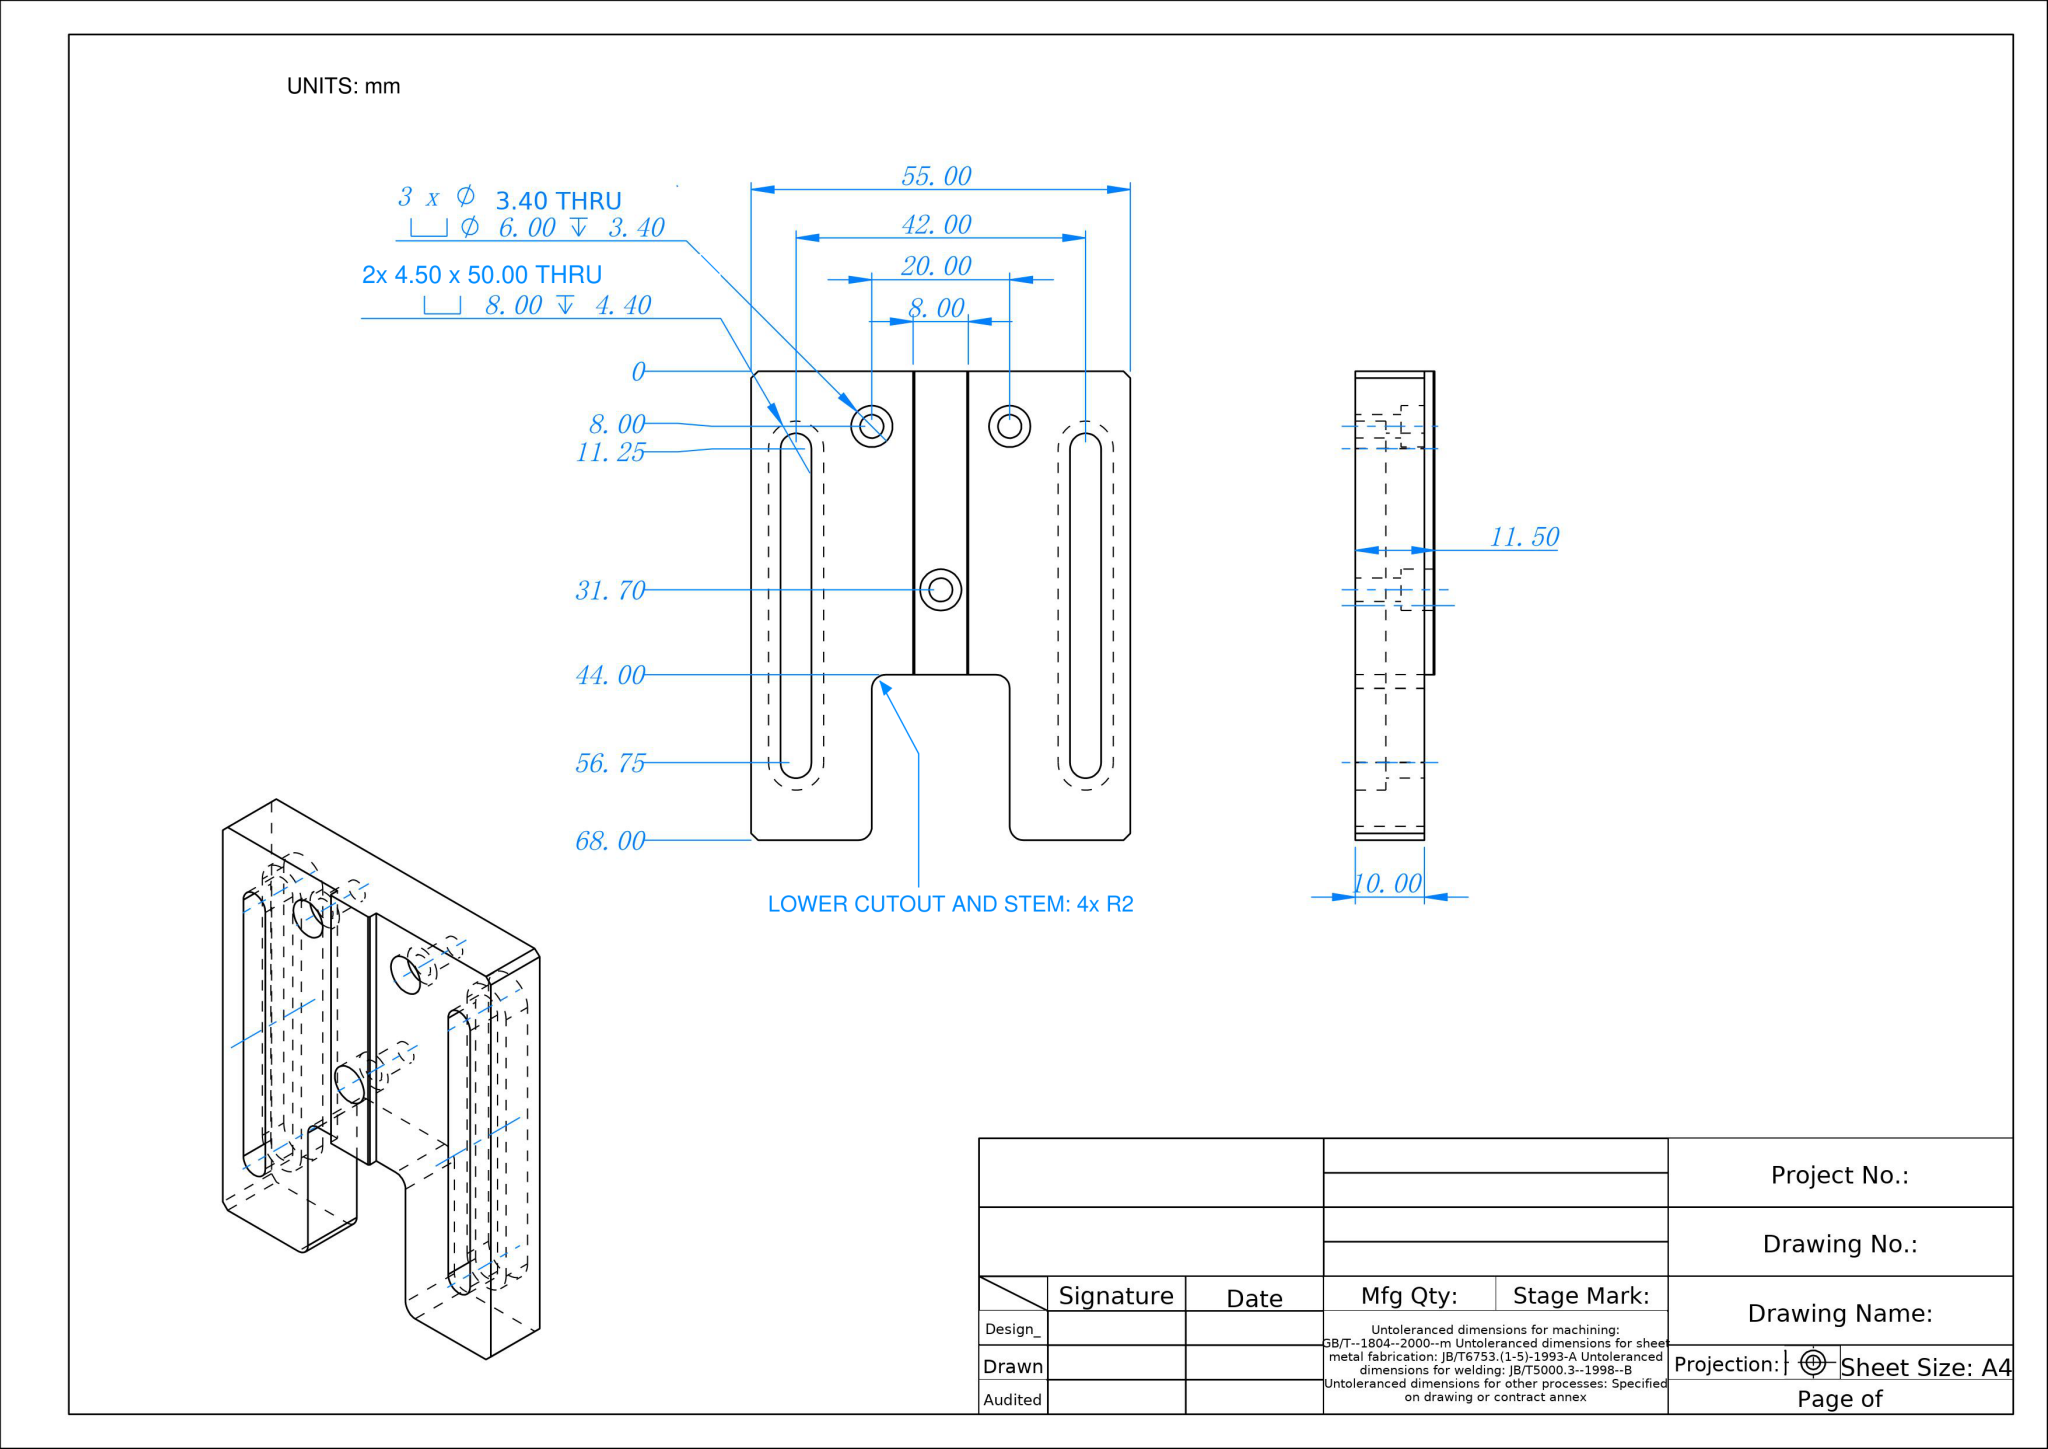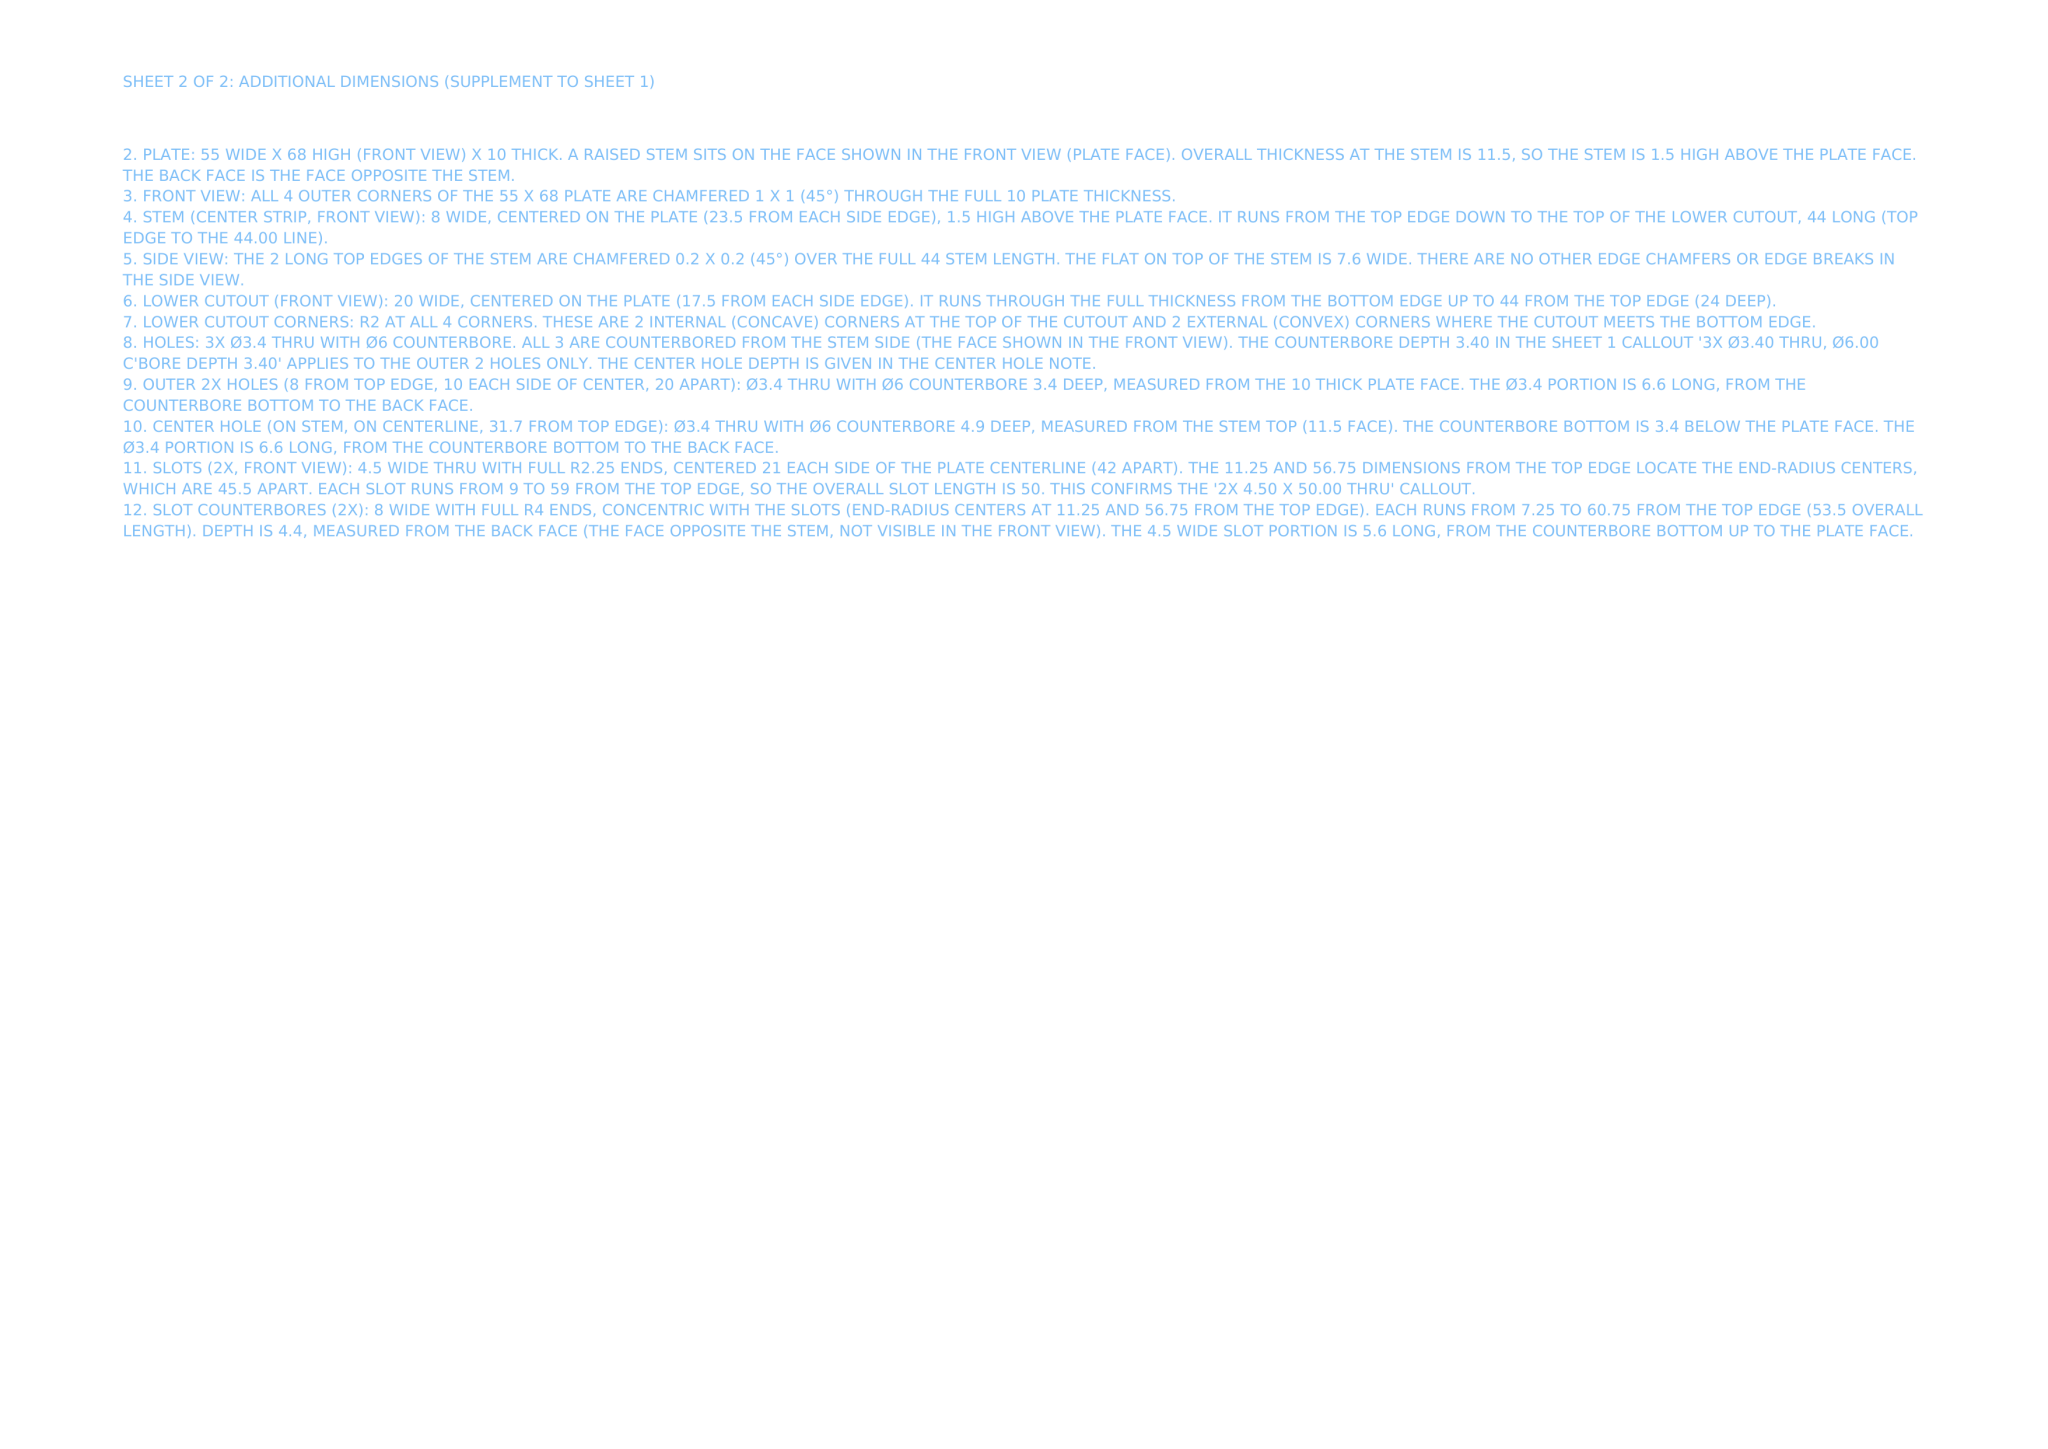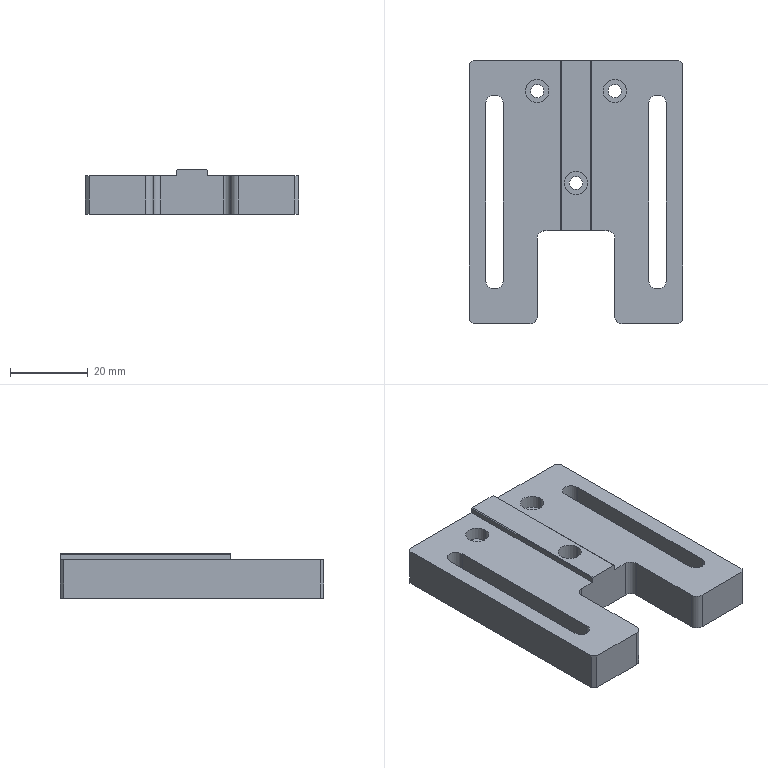Part | NX | mm | 1 solid | 57 faces | box 55 x 68 x 11.5 mm | volume 26479 mm3 | plane 33 | cylinder 24 | commonest cylinder face diameters 6 x6 3.4 x6 4.5 x4 8 x4 4 x4